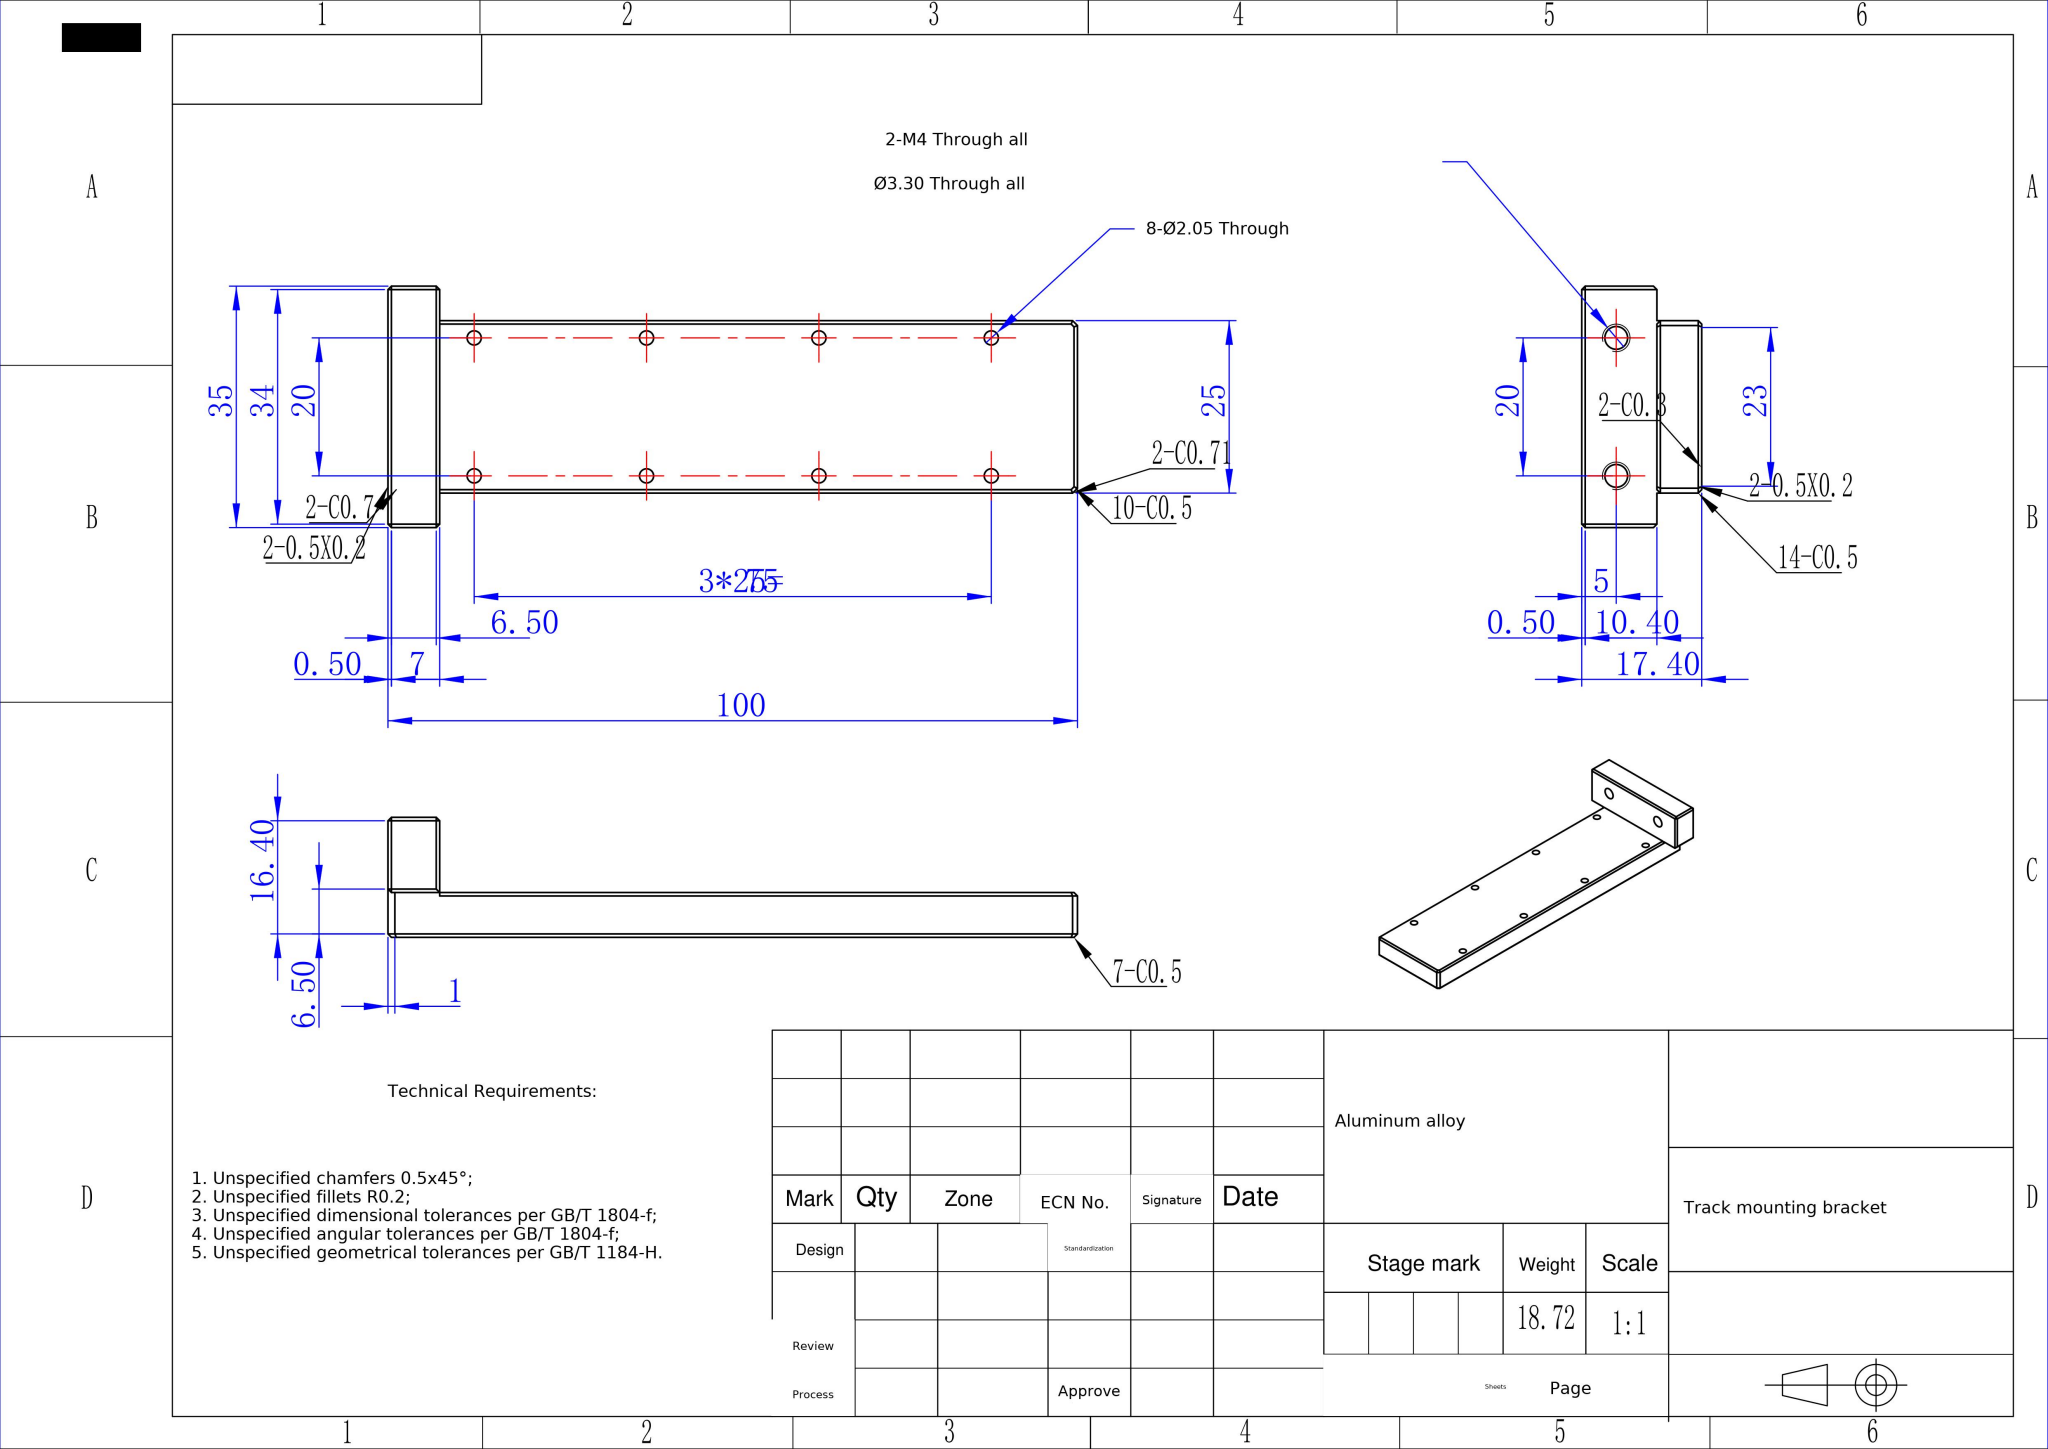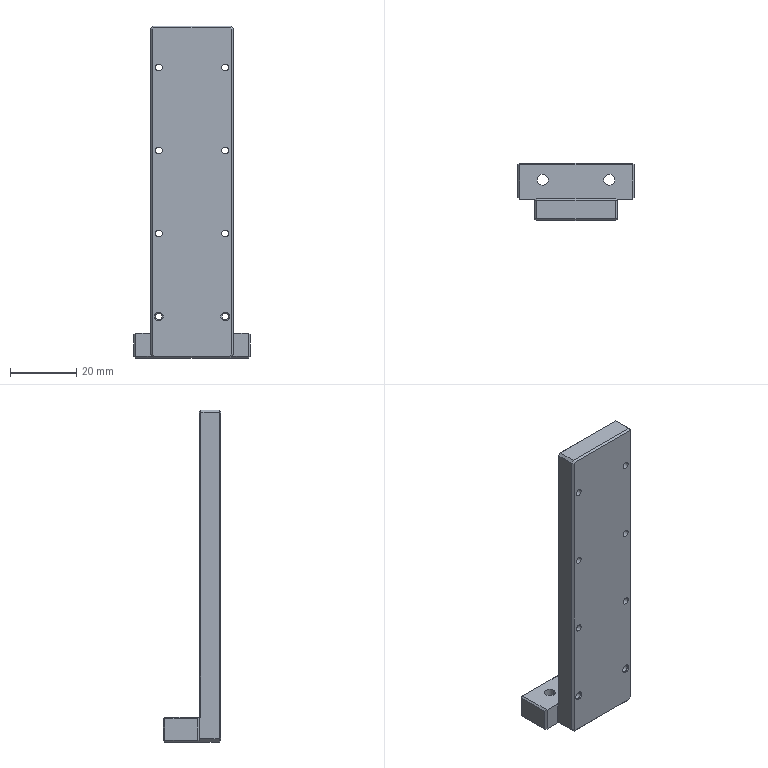Part | SolidWorks | mm | material Aluminum alloy | 1 solid | 75 faces | box 35 x 17.4 x 100 mm | volume 18724 mm3 | plane 47 | cylinder 20 | cone 8 | commonest cylinder face diameters 2.05 x16 3.3 x4